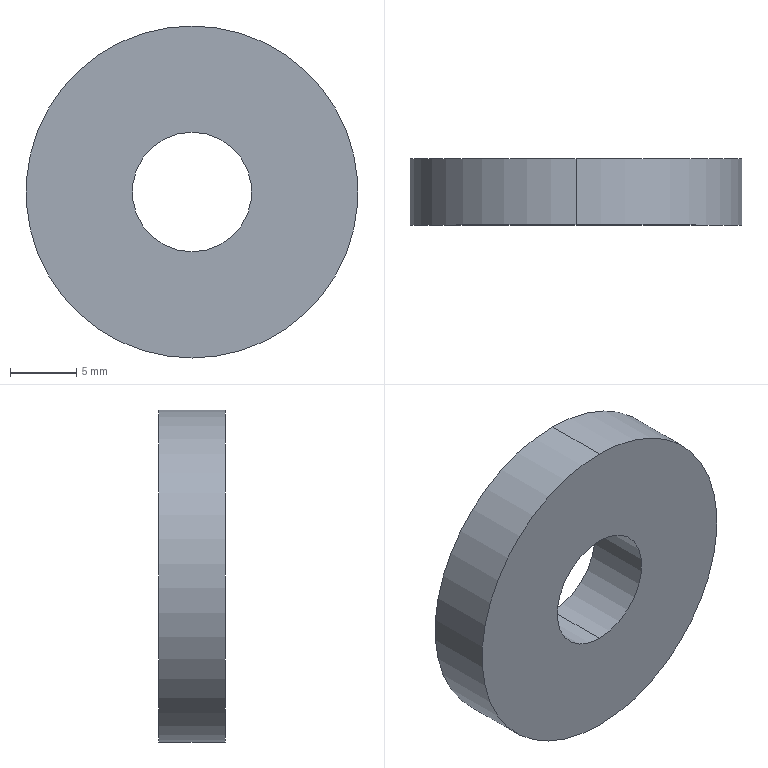Component | SolidWorks | F12529-M1073-2 | 1 solid | 6 faces | box 25 x 5 x 25 mm | volume 2136 mm3 | cylinder 4 | plane 2 | commonest cylinder face diameters 9 x2 25 x2
build123d program:
from build123d import *

# Parameters (mm, degrees)
SKETCH1_R           = 12.5
SKETCH1_R_2         = 4.5
BOSS_EXTRUDE1_DEPTH = 5


with BuildPart() as part:
    # Sketch1 → Boss-Extrude1 (new body)
    with BuildSketch(Plane(origin=(0, 0, 0), x_dir=(1, 0, 0), z_dir=(0, 1, 0))):
        with Locations(Location((0, 0, 0), (0, 0, 270))):
            Circle(SKETCH1_R)
        with Locations(Location((0, 0, 0), (0, 0, 270))):
            Circle(SKETCH1_R_2, mode=Mode.SUBTRACT)
    extrude(amount=BOSS_EXTRUDE1_DEPTH)


solid = part.part

# Placed as in the assembly
solid = solid.moved(Location((-37.5, -10, -20), (0, 0, 0)))
STEP:
#1=COLOUR_RGB('',0.7922,0.8196,0.9333);
#2=FILL_AREA_STYLE_COLOUR('',#1);
#3=FILL_AREA_STYLE('',(#2));
#4=SURFACE_STYLE_FILL_AREA(#3);
#5=SURFACE_SIDE_STYLE('',(#4));
#6=SURFACE_STYLE_USAGE(.BOTH.,#5);
#7=PRESENTATION_STYLE_ASSIGNMENT((#6));
#8=CARTESIAN_POINT('',(-1.476,-0.1969,-0.9646));
#9=VERTEX_POINT('',#8);
#10=CARTESIAN_POINT('',(-1.476,-0.1969,-0.6102));
#11=VERTEX_POINT('',#10);
#12=CARTESIAN_POINT('',(-1.476,-0.1969,-0.7874));
#13=DIRECTION('',(0.,1.,0.));
#14=DIRECTION('',(0.,0.,1.));
#15=AXIS2_PLACEMENT_3D('',#12,#13,#14);
#16=CIRCLE('',#15,0.1772);
#17=EDGE_CURVE('',#9,#11,#16,.T.);
#18=ORIENTED_EDGE('',*,*,#17,.T.);
#19=CARTESIAN_POINT('',(-1.476,-0.3937,-0.6102));
#20=VERTEX_POINT('',#19);
#21=CARTESIAN_POINT('',(-1.476,-0.1969,-0.6102));
#22=DIRECTION('',(0.,-1.,0.));
#23=VECTOR('',#22,39.37);
#24=LINE('',#21,#23);
#25=EDGE_CURVE('',#11,#20,#24,.T.);
#26=ORIENTED_EDGE('',*,*,#25,.T.);
#27=CARTESIAN_POINT('',(-1.476,-0.3937,-0.9646));
#28=VERTEX_POINT('',#27);
#29=CARTESIAN_POINT('',(-1.476,-0.3937,-0.7874));
#30=DIRECTION('',(0.,1.,0.));
#31=DIRECTION('',(0.,0.,1.));
#32=AXIS2_PLACEMENT_3D('',#29,#30,#31);
#33=CIRCLE('',#32,0.1772);
#34=EDGE_CURVE('',#28,#20,#33,.T.);
#35=ORIENTED_EDGE('',*,*,#34,.F.);
#36=CARTESIAN_POINT('',(-1.476,-0.1969,-0.9646));
#37=DIRECTION('',(0.,-1.,0.));
#38=VECTOR('',#37,39.37);
#39=LINE('',#36,#38);
#40=EDGE_CURVE('',#9,#28,#39,.T.);
#41=ORIENTED_EDGE('',*,*,#40,.F.);
#42=EDGE_LOOP('',(#18,#26,#35,#41));
#43=FACE_OUTER_BOUND('',#42,.T.);
#44=CARTESIAN_POINT('',(-1.476,-0.1969,-0.7874));
#45=DIRECTION('',(0.,-1.,0.));
#46=DIRECTION('',(0.,0.,-1.));
#47=AXIS2_PLACEMENT_3D('',#44,#45,#46);
#48=CYLINDRICAL_SURFACE('',#47,0.1772);
#49=ADVANCED_FACE('',(#43),#48,.F.);
#50=CARTESIAN_POINT('',(-1.476,-0.1969,-0.2953));
#51=VERTEX_POINT('',#50);
#52=CARTESIAN_POINT('',(-1.476,-0.1969,-1.28));
#53=VERTEX_POINT('',#52);
#54=CARTESIAN_POINT('',(-1.476,-0.1969,-0.7874));
#55=DIRECTION('',(0.,1.,0.));
#56=DIRECTION('',(0.,0.,1.));
#57=AXIS2_PLACEMENT_3D('',#54,#55,#56);
#58=CIRCLE('',#57,0.4921);
#59=EDGE_CURVE('',#51,#53,#58,.T.);
#60=ORIENTED_EDGE('',*,*,#59,.F.);
#61=CARTESIAN_POINT('',(-1.476,-0.3937,-0.2953));
#62=VERTEX_POINT('',#61);
#63=CARTESIAN_POINT('',(-1.476,-0.1969,-0.2953));
#64=DIRECTION('',(0.,-1.,0.));
#65=VECTOR('',#64,39.37);
#66=LINE('',#63,#65);
#67=EDGE_CURVE('',#51,#62,#66,.T.);
#68=ORIENTED_EDGE('',*,*,#67,.T.);
#69=CARTESIAN_POINT('',(-1.476,-0.3937,-1.28));
#70=VERTEX_POINT('',#69);
#71=CARTESIAN_POINT('',(-1.476,-0.3937,-0.7874));
#72=DIRECTION('',(0.,1.,0.));
#73=DIRECTION('',(0.,0.,1.));
#74=AXIS2_PLACEMENT_3D('',#71,#72,#73);
#75=CIRCLE('',#74,0.4921);
#76=EDGE_CURVE('',#62,#70,#75,.T.);
#77=ORIENTED_EDGE('',*,*,#76,.T.);
#78=CARTESIAN_POINT('',(-1.476,-0.1969,-1.28));
#79=DIRECTION('',(0.,-1.,0.));
#80=VECTOR('',#79,39.37);
#81=LINE('',#78,#80);
#82=EDGE_CURVE('',#53,#70,#81,.T.);
#83=ORIENTED_EDGE('',*,*,#82,.F.);
#84=EDGE_LOOP('',(#60,#68,#77,#83));
#85=FACE_OUTER_BOUND('',#84,.T.);
#86=CARTESIAN_POINT('',(-1.476,-0.1969,-0.7874));
#87=DIRECTION('',(0.,-1.,0.));
#88=DIRECTION('',(0.,0.,-1.));
#89=AXIS2_PLACEMENT_3D('',#86,#87,#88);
#90=CYLINDRICAL_SURFACE('',#89,0.4921);
#91=ADVANCED_FACE('',(#85),#90,.T.);
#92=CARTESIAN_POINT('',(-1.476,-0.1969,-0.7874));
#93=DIRECTION('',(0.,1.,0.));
#94=DIRECTION('',(0.,0.,1.));
#95=AXIS2_PLACEMENT_3D('',#92,#93,#94);
#96=CIRCLE('',#95,0.4921);
#97=EDGE_CURVE('',#53,#51,#96,.T.);
#98=ORIENTED_EDGE('',*,*,#97,.T.);
#99=ORIENTED_EDGE('',*,*,#59,.T.);
#100=EDGE_LOOP('',(#98,#99));
#101=FACE_OUTER_BOUND('',#100,.T.);
#102=ORIENTED_EDGE('',*,*,#17,.F.);
#103=CARTESIAN_POINT('',(-1.476,-0.1969,-0.7874));
#104=DIRECTION('',(0.,1.,0.));
#105=DIRECTION('',(0.,0.,1.));
#106=AXIS2_PLACEMENT_3D('',#103,#104,#105);
#107=CIRCLE('',#106,0.1772);
#108=EDGE_CURVE('',#11,#9,#107,.T.);
#109=ORIENTED_EDGE('',*,*,#108,.F.);
#110=EDGE_LOOP('',(#102,#109));
#111=FACE_BOUND('',#110,.T.);
#112=CARTESIAN_POINT('',(-1.476,-0.1969,-0.7874));
#113=DIRECTION('',(0.,1.,0.));
#114=DIRECTION('',(0.,0.,1.));
#115=AXIS2_PLACEMENT_3D('',#112,#113,#114);
#116=PLANE('',#115);
#117=ADVANCED_FACE('',(#101,#111),#116,.T.);
#118=CARTESIAN_POINT('',(-1.476,-0.3937,-0.7874));
#119=DIRECTION('',(0.,1.,0.));
#120=DIRECTION('',(0.,0.,1.));
#121=AXIS2_PLACEMENT_3D('',#118,#119,#120);
#122=CIRCLE('',#121,0.4921);
#123=EDGE_CURVE('',#70,#62,#122,.T.);
#124=ORIENTED_EDGE('',*,*,#123,.F.);
#125=ORIENTED_EDGE('',*,*,#76,.F.);
#126=EDGE_LOOP('',(#124,#125));
#127=FACE_OUTER_BOUND('',#126,.T.);
#128=ORIENTED_EDGE('',*,*,#34,.T.);
#129=CARTESIAN_POINT('',(-1.476,-0.3937,-0.7874));
#130=DIRECTION('',(0.,1.,0.));
#131=DIRECTION('',(0.,0.,1.));
#132=AXIS2_PLACEMENT_3D('',#129,#130,#131);
#133=CIRCLE('',#132,0.1772);
#134=EDGE_CURVE('',#20,#28,#133,.T.);
#135=ORIENTED_EDGE('',*,*,#134,.T.);
#136=EDGE_LOOP('',(#128,#135));
#137=FACE_BOUND('',#136,.T.);
#138=CARTESIAN_POINT('',(-1.476,-0.3937,-0.7874));
#139=DIRECTION('',(0.,1.,0.));
#140=DIRECTION('',(0.,0.,1.));
#141=AXIS2_PLACEMENT_3D('',#138,#139,#140);
#142=PLANE('',#141);
#143=ADVANCED_FACE('',(#127,#137),#142,.F.);
#144=ORIENTED_EDGE('',*,*,#67,.F.);
#145=ORIENTED_EDGE('',*,*,#97,.F.);
#146=ORIENTED_EDGE('',*,*,#82,.T.);
#147=ORIENTED_EDGE('',*,*,#123,.T.);
#148=EDGE_LOOP('',(#144,#145,#146,#147));
#149=FACE_OUTER_BOUND('',#148,.T.);
#150=CARTESIAN_POINT('',(-1.476,-0.1969,-0.7874));
#151=DIRECTION('',(0.,-1.,0.));
#152=DIRECTION('',(0.,0.,-1.));
#153=AXIS2_PLACEMENT_3D('',#150,#151,#152);
#154=CYLINDRICAL_SURFACE('',#153,0.4921);
#155=ADVANCED_FACE('',(#149),#154,.T.);
#156=ORIENTED_EDGE('',*,*,#25,.F.);
#157=ORIENTED_EDGE('',*,*,#108,.T.);
#158=ORIENTED_EDGE('',*,*,#40,.T.);
#159=ORIENTED_EDGE('',*,*,#134,.F.);
#160=EDGE_LOOP('',(#156,#157,#158,#159));
#161=FACE_OUTER_BOUND('',#160,.T.);
#162=CARTESIAN_POINT('',(-1.476,-0.1969,-0.7874));
#163=DIRECTION('',(0.,-1.,0.));
#164=DIRECTION('',(0.,0.,-1.));
#165=AXIS2_PLACEMENT_3D('',#162,#163,#164);
#166=CYLINDRICAL_SURFACE('',#165,0.1772);
#167=ADVANCED_FACE('',(#161),#166,.F.);
#168=CLOSED_SHELL('',(#49,#91,#117,#143,#155,#167));
#169=MANIFOLD_SOLID_BREP('',#168);
#170=STYLED_ITEM('',(#7),#169);
#171=PRESENTATION_LAYER_ASSIGNMENT('','',(#170));
#172=(LENGTH_UNIT()NAMED_UNIT(*)SI_UNIT($,.METRE.));
#173=LENGTH_MEASURE_WITH_UNIT(LENGTH_MEASURE(0.0254),#172);
#174=DIMENSIONAL_EXPONENTS(1.,0.,0.,0.,0.,0.,0.);
#175=(CONVERSION_BASED_UNIT('',#173)LENGTH_UNIT()NAMED_UNIT(#174));
#176=UNCERTAINTY_MEASURE_WITH_UNIT(LENGTH_MEASURE(0.00001),#175,'','');
#177=(NAMED_UNIT(*)PLANE_ANGLE_UNIT()SI_UNIT($,.RADIAN.));
#178=(NAMED_UNIT(*)SI_UNIT($,.STERADIAN.)SOLID_ANGLE_UNIT());
#179=(GEOMETRIC_REPRESENTATION_CONTEXT(3)GLOBAL_UNCERTAINTY_ASSIGNED_CONTEXT((#176))GLOBAL_UNIT_ASSIGNED_CONTEXT((#175,#177,#178))REPRESENTATION_CONTEXT('',''));
#180=MECHANICAL_DESIGN_GEOMETRIC_PRESENTATION_REPRESENTATION('',(#170),#179);
#181=CARTESIAN_POINT('',(0.,0.,0.));
#182=DIRECTION('',(0.,0.,1.));
#183=DIRECTION('',(1.,0.,0.));
#184=AXIS2_PLACEMENT_3D('',#181,#182,#183);
#185=(LENGTH_UNIT()NAMED_UNIT(*)SI_UNIT($,.METRE.));
#186=LENGTH_MEASURE_WITH_UNIT(LENGTH_MEASURE(0.0254),#185);
#187=DIMENSIONAL_EXPONENTS(1.,0.,0.,0.,0.,0.,0.);
#188=(CONVERSION_BASED_UNIT('',#186)LENGTH_UNIT()NAMED_UNIT(#187));
#189=UNCERTAINTY_MEASURE_WITH_UNIT(LENGTH_MEASURE(0.00001),#188,'','');
#190=(NAMED_UNIT(*)PLANE_ANGLE_UNIT()SI_UNIT($,.RADIAN.));
#191=(NAMED_UNIT(*)SI_UNIT($,.STERADIAN.)SOLID_ANGLE_UNIT());
#192=(GEOMETRIC_REPRESENTATION_CONTEXT(3)GLOBAL_UNCERTAINTY_ASSIGNED_CONTEXT((#189))GLOBAL_UNIT_ASSIGNED_CONTEXT((#188,#190,#191))REPRESENTATION_CONTEXT('',''));
#193=ADVANCED_BREP_SHAPE_REPRESENTATION('',(#169,#184),#192);